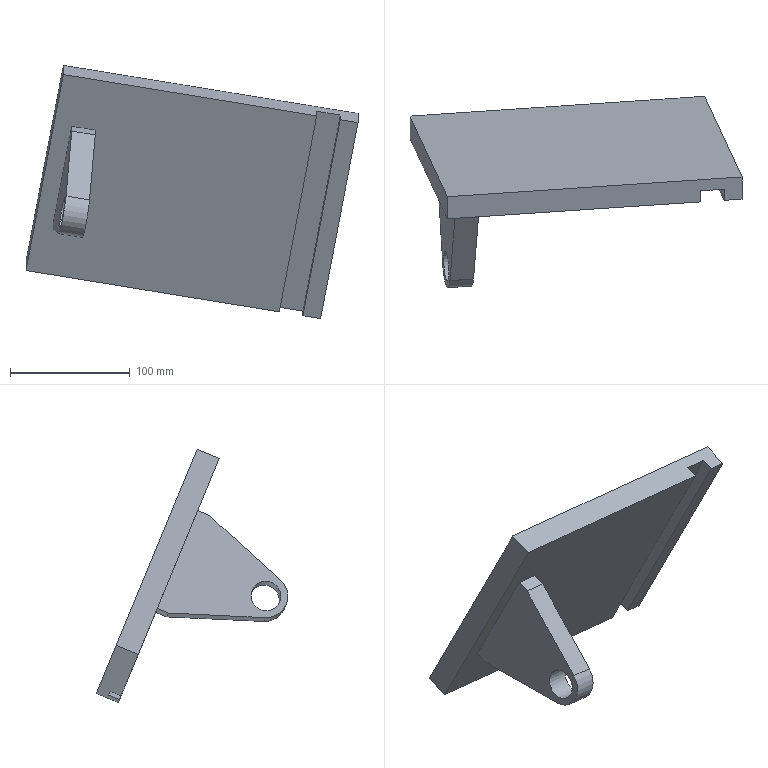Component | NX | 1 | 2 solids | 19 faces | volume 973186 mm3 | plane 17 | cylinder 2 | commonest cylinder face diameters 36.69 x1 25 x1